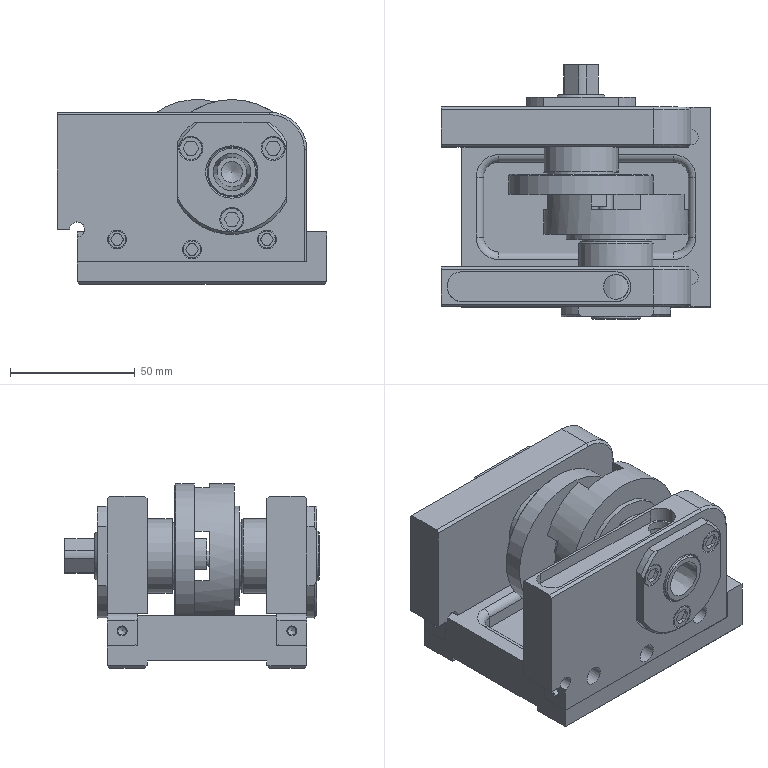Assembly | NX | mm | 25 component files | 25 solids | 563 faces | box 108 x 102 x 74 mm | volume 345953 mm3 | plane 263 | cylinder 204 | cone 87 | torus 9 | commonest cylinder face diameters 2 x72 7.5 x14 4.3 x14 3.3 x14 6 x13 3.242 x12 12 x7 8.907 x6
Bill of materials:
unnamed part 1 | 1 |  | Turned part with a thin circular disc flange. A stepped cylindrical shaft sticks out from one face and ends in a narrower end section. A small off-center pin and a bent raised feature stand on the opposite face.
unnamed part 2 | 1 |  | Thick rectangular plate with one large rounded corner and a large central round through-bore. Three small countersunk holes surround the bore and three through-holes run along the lower edge. There is a semicircular notch at one lower corner, a stepped lower edge, and a long slot cut into the top edge face.
unnamed part 3 | 1 |  | Flanged bushing: a cylindrical sleeve with a central through-bore on a flange that is round with flats cut on its sides. The flange has three countersunk holes, and the sleeve has a radial cross hole in its wall.
unnamed part 4 | 6 |  | Headed pin: a short cylindrical head on a plain cylindrical shank, with chamfered edges.
unnamed part 5 | 1 |  | Flanged sleeve: a thin-walled cylindrical tube on a flange that is round with flats cut on its sides. The flange has three plain through-holes. The bore is stepped (counterbored) at the open end, and there is an undercut next to the flange.
unnamed part 6 | 1 |  | Thick rectangular plate with one large rounded corner and a large central round through-bore. Three small holes run along the lower edge, with a semicircular notch at one lower corner and a step along the bottom edge.
unnamed part 7 | 1 |  | Rectangular block with a shallow rounded-rectangle pocket in the top face and a lower ledge along one long side. Small holes are drilled in the side faces and larger cross holes in the end faces. A relief channel runs along the underside between two feet.
unnamed part 8 | 6 |  | Plain flat ring/washer: a thin annulus with a central round hole.
unnamed part 9 | 6 |  | Countersunk (conical) head pin: a cone-shaped head on a plain cylindrical shank with a chamfered end.
unnamed part 10 | 1 |  | Stepped turned part: a large disc with rectangular notches in its rim, then a smaller step and a collar, then a hollow cylindrical spigot. A central blind bore ends in a conical drill-point bottom.
Mates:
1. fix | Base 1 component
2. concentric | Base 1 edge | Left_Plate 1 edge
3. parallel | Left_Plate 1 face | Base 1 face
4. concentric | Left_Plate 1 edge | Geneva_Sleeve 1 edge
5. parallel | Geneva_Sleeve 1 face | Left_Plate 1 face
6. concentric | Geneva_Shaft 1 edge | Geneva_Sleeve 1 edge
7. concentric | Right_Plate 1 arc | Base 1 edge
8. parallel | Right_Plate 1 face | Base 1 face
9. concentric | Right_Plate 1 edge | Indexing_Sleeve 1 edge
10. parallel | Indexing_Sleeve 1 face | Right_Plate 1 face
11. concentric | Indexing_Shaft 1 edge | Indexing_Sleeve 1 edge
12. concentric | Spring_Washer 6 arc | Left_Plate 1 edge
13. concentric | Spring_Washer 5 arc | Left_Plate 1 edge
14. concentric | Spring_Washer 4 arc | Left_Plate 1 edge
15. concentric | Spring_Washer 3 arc | Right_Plate 1 edge
16. concentric | Spring_Washer 2 arc | Right_Plate 1 edge
17. concentric | Spring_Washer 1 arc | Right_Plate 1 edge
18. concentric | Hex_Cap_Screw 6 arc | Spring_Washer 6 edge
19. parallel | Hex_Cap_Screw 6 face | Left_Plate 1 face
20. concentric | Hex_Cap_Screw 5 arc | Spring_Washer 5 edge
21. parallel | Hex_Cap_Screw 5 face | Left_Plate 1 face
22. concentric | Hex_Cap_Screw 4 arc | Spring_Washer 4 edge
23. parallel | Hex_Cap_Screw 4 face | Left_Plate 1 face
24. concentric | Hex_Cap_Screw 3 arc | Spring_Washer 3 edge
25. parallel | Hex_Cap_Screw 3 face | Right_Plate 1 face
26. concentric | Hex_Cap_Screw 2 arc | Spring_Washer 2 edge
27. parallel | Hex_Cap_Screw 2 face | Right_Plate 1 face
28. concentric | Hex_Cap_Screw 1 arc | Spring_Washer 1 edge
29. parallel | Hex_Cap_Screw 1 face | Right_Plate 1 face
30. concentric | Hex_Flat_Screw 6 edge | Geneva_Sleeve 1 edge
31. parallel | Hex_Flat_Screw 6 face | Geneva_Sleeve 1 face
32. fix | assembly component
33. bond | Hex_Flat_Screw 6 component | assembly component
34. bond | Hex_Flat_Screw 5 component | assembly component
35. bond | Hex_Flat_Screw 4 component | assembly component
36. circular | assembly datumaxis | assembly cartesiancoordinatesystem | assembly cartesiancoordinatesystem | assembly cartesiancoordinatesystem
37. concentric | Hex_Flat_Screw 3 edge | Indexing_Sleeve 1 edge
38. parallel | Hex_Flat_Screw 3 face | Right_Plate 1 face
39. fix | assembly component
40. bond | Hex_Flat_Screw 3 component | assembly component
41. bond | Hex_Flat_Screw 2 component | assembly component
42. bond | Hex_Flat_Screw 1 component | assembly component
43. circular | assembly datumaxis | assembly cartesiancoordinatesystem | assembly cartesiancoordinatesystem | assembly cartesiancoordinatesystem